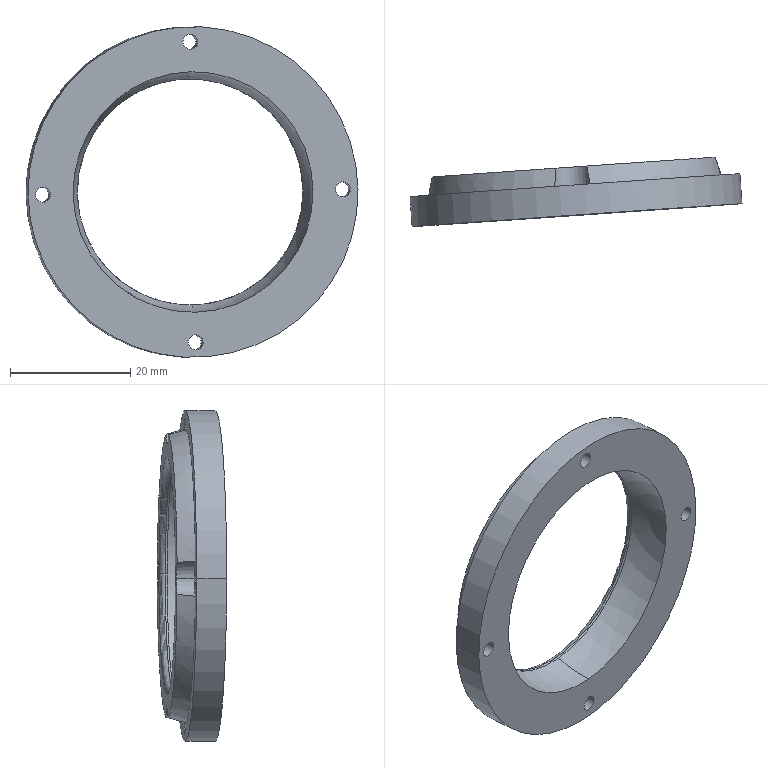Component | SolidWorks | ClampingMechanism-1_BallJointFixed-1 | 1 solid | 28 faces | box 55.21 x 11.53 x 55 mm | volume 7588 mm3 | cylinder 15 | sphere 6 | torus 4 | plane 3 | commonest cylinder face diameters 2.5 x8 6 x5 55 x2
STEP:
#1=COLOUR_RGB('',0.7922,0.8196,0.9333);
#2=FILL_AREA_STYLE_COLOUR('',#1);
#3=FILL_AREA_STYLE('',(#2));
#4=SURFACE_STYLE_FILL_AREA(#3);
#5=SURFACE_SIDE_STYLE('',(#4));
#6=SURFACE_STYLE_USAGE(.BOTH.,#5);
#7=PRESENTATION_STYLE_ASSIGNMENT((#6));
#8=CARTESIAN_POINT('',(1.976,-7.995,-21.39));
#9=VERTEX_POINT('',#8);
#10=CARTESIAN_POINT('',(1.934,-7.959,-21.391));
#11=VERTEX_POINT('',#10);
#12=CARTESIAN_POINT('',(1.937,-7.998,-21.391));
#13=DIRECTION('',(-0.01767,-0.001232,0.9998));
#14=DIRECTION('',(0.9998,0.,0.01767));
#15=AXIS2_PLACEMENT_3D('',#12,#13,#14);
#16=CIRCLE('',#15,0.03937);
#17=EDGE_CURVE('',#9,#11,#16,.T.);
#18=ORIENTED_EDGE('',*,*,#17,.F.);
#19=CARTESIAN_POINT('',(3.452,-7.892,-21.364));
#20=VERTEX_POINT('',#19);
#21=CARTESIAN_POINT('',(2.714,-7.944,-21.377));
#22=DIRECTION('',(0.06956,-0.9976,-0.));
#23=DIRECTION('',(0.9976,0.06956,0.));
#24=AXIS2_PLACEMENT_3D('',#21,#22,#23);
#25=CIRCLE('',#24,0.7401);
#26=EDGE_CURVE('',#9,#20,#25,.T.);
#27=ORIENTED_EDGE('',*,*,#26,.T.);
#28=CARTESIAN_POINT('',(3.489,-7.85,-21.363));
#29=VERTEX_POINT('',#28);
#30=CARTESIAN_POINT('',(3.492,-7.89,-21.363));
#31=DIRECTION('',(0.01767,0.001232,-0.9998));
#32=DIRECTION('',(-0.9998,0.,-0.01767));
#33=AXIS2_PLACEMENT_3D('',#30,#31,#32);
#34=CIRCLE('',#33,0.03937);
#35=EDGE_CURVE('',#20,#29,#34,.T.);
#36=ORIENTED_EDGE('',*,*,#35,.T.);
#37=CARTESIAN_POINT('',(2.711,-7.905,-21.377));
#38=DIRECTION('',(0.06956,-0.9976,-0.));
#39=DIRECTION('',(0.9974,0.06955,0.01772));
#40=AXIS2_PLACEMENT_3D('',#37,#38,#39);
#41=CIRCLE('',#40,0.7795);
#42=EDGE_CURVE('',#11,#29,#41,.T.);
#43=ORIENTED_EDGE('',*,*,#42,.F.);
#44=EDGE_LOOP('',(#18,#27,#36,#43));
#45=FACE_OUTER_BOUND('',#44,.T.);
#46=CARTESIAN_POINT('',(2.714,-7.944,-21.377));
#47=DIRECTION('',(0.06956,-0.9976,-0.));
#48=DIRECTION('',(0.9974,0.06955,0.01772));
#49=AXIS2_PLACEMENT_3D('',#46,#47,#48);
#50=TOROIDAL_SURFACE('',#49,0.7795,0.03937);
#51=ADVANCED_FACE('',(#45),#50,.T.);
#52=ORIENTED_EDGE('',*,*,#35,.F.);
#53=CARTESIAN_POINT('',(2.714,-7.944,-21.377));
#54=DIRECTION('',(0.06956,-0.9976,-0.));
#55=DIRECTION('',(0.9976,0.06956,0.));
#56=AXIS2_PLACEMENT_3D('',#53,#54,#55);
#57=CIRCLE('',#56,0.7401);
#58=EDGE_CURVE('',#20,#9,#57,.T.);
#59=ORIENTED_EDGE('',*,*,#58,.T.);
#60=ORIENTED_EDGE('',*,*,#17,.T.);
#61=CARTESIAN_POINT('',(2.711,-7.905,-21.377));
#62=DIRECTION('',(0.06956,-0.9976,-0.));
#63=DIRECTION('',(0.9974,0.06955,0.01772));
#64=AXIS2_PLACEMENT_3D('',#61,#62,#63);
#65=CIRCLE('',#64,0.7795);
#66=EDGE_CURVE('',#29,#11,#65,.T.);
#67=ORIENTED_EDGE('',*,*,#66,.F.);
#68=EDGE_LOOP('',(#52,#59,#60,#67));
#69=FACE_OUTER_BOUND('',#68,.T.);
#70=CARTESIAN_POINT('',(2.714,-7.944,-21.377));
#71=DIRECTION('',(0.06956,-0.9976,-0.));
#72=DIRECTION('',(0.9974,0.06955,0.01772));
#73=AXIS2_PLACEMENT_3D('',#70,#71,#72);
#74=TOROIDAL_SURFACE('',#73,0.7795,0.03937);
#75=ADVANCED_FACE('',(#69),#74,.T.);
#76=ORIENTED_EDGE('',*,*,#58,.F.);
#77=CARTESIAN_POINT('',(3.456,-7.905,-21.364));
#78=VERTEX_POINT('',#77);
#79=CARTESIAN_POINT('',(3.492,-7.89,-21.363));
#80=DIRECTION('',(0.01767,0.001232,-0.9998));
#81=DIRECTION('',(-0.9998,0.,-0.01767));
#82=AXIS2_PLACEMENT_3D('',#79,#80,#81);
#83=CIRCLE('',#82,0.03937);
#84=EDGE_CURVE('',#78,#20,#83,.T.);
#85=ORIENTED_EDGE('',*,*,#84,.F.);
#86=CARTESIAN_POINT('',(2.702,-7.958,-20.635));
#87=VERTEX_POINT('',#86);
#88=CARTESIAN_POINT('',(2.715,-7.957,-21.377));
#89=DIRECTION('',(-0.06956,0.9976,0.));
#90=DIRECTION('',(0.9974,0.06955,0.01772));
#91=AXIS2_PLACEMENT_3D('',#88,#89,#90);
#92=CIRCLE('',#91,0.7424);
#93=EDGE_CURVE('',#87,#78,#92,.T.);
#94=ORIENTED_EDGE('',*,*,#93,.F.);
#95=CARTESIAN_POINT('',(1.975,-8.009,-21.39));
#96=VERTEX_POINT('',#95);
#97=CARTESIAN_POINT('',(2.715,-7.957,-21.377));
#98=DIRECTION('',(-0.06956,0.9976,0.));
#99=DIRECTION('',(0.9974,0.06955,0.01772));
#100=AXIS2_PLACEMENT_3D('',#97,#98,#99);
#101=CIRCLE('',#100,0.7424);
#102=EDGE_CURVE('',#96,#87,#101,.T.);
#103=ORIENTED_EDGE('',*,*,#102,.F.);
#104=CARTESIAN_POINT('',(1.937,-7.998,-21.391));
#105=DIRECTION('',(-0.01767,-0.001232,0.9998));
#106=DIRECTION('',(0.9998,0.,0.01767));
#107=AXIS2_PLACEMENT_3D('',#104,#105,#106);
#108=CIRCLE('',#107,0.03937);
#109=EDGE_CURVE('',#96,#9,#108,.T.);
#110=ORIENTED_EDGE('',*,*,#109,.T.);
#111=EDGE_LOOP('',(#76,#85,#94,#103,#110));
#112=FACE_OUTER_BOUND('',#111,.T.);
#113=CARTESIAN_POINT('',(2.714,-7.944,-21.377));
#114=DIRECTION('',(0.06956,-0.9976,-0.));
#115=DIRECTION('',(0.9974,0.06955,0.01772));
#116=AXIS2_PLACEMENT_3D('',#113,#114,#115);
#117=TOROIDAL_SURFACE('',#116,0.7795,0.03937);
#118=ADVANCED_FACE('',(#112),#117,.T.);
#119=CARTESIAN_POINT('',(1.848,-7.965,-21.392));
#120=VERTEX_POINT('',#119);
#121=CARTESIAN_POINT('',(1.785,-7.969,-21.29));
#122=VERTEX_POINT('',#121);
#123=CARTESIAN_POINT('',(1.73,-7.973,-21.394));
#124=DIRECTION('',(0.06956,-0.9976,-0.));
#125=DIRECTION('',(0.9974,0.06955,0.01772));
#126=AXIS2_PLACEMENT_3D('',#123,#124,#125);
#127=CIRCLE('',#126,0.1181);
#128=EDGE_CURVE('',#120,#122,#127,.T.);
#129=ORIENTED_EDGE('',*,*,#128,.F.);
#130=CARTESIAN_POINT('',(1.856,-8.083,-21.392));
#131=VERTEX_POINT('',#130);
#132=CARTESIAN_POINT('',(1.828,-7.69,-21.392));
#133=DIRECTION('',(0.06956,-0.9976,-0.));
#134=VECTOR('',#133,39.37);
#135=LINE('',#132,#134);
#136=EDGE_CURVE('',#120,#131,#135,.T.);
#137=ORIENTED_EDGE('',*,*,#136,.T.);
#138=CARTESIAN_POINT('',(1.763,-8.089,-21.279));
#139=VERTEX_POINT('',#138);
#140=CARTESIAN_POINT('',(1.738,-8.091,-21.394));
#141=DIRECTION('',(-0.06956,0.9976,0.));
#142=DIRECTION('',(-0.9974,-0.06955,-0.01772));
#143=AXIS2_PLACEMENT_3D('',#140,#141,#142);
#144=CIRCLE('',#143,0.1181);
#145=EDGE_CURVE('',#139,#131,#144,.T.);
#146=ORIENTED_EDGE('',*,*,#145,.F.);
#147=CARTESIAN_POINT('',(1.763,-8.089,-21.279));
#148=CARTESIAN_POINT('',(1.768,-8.048,-21.28));
#149=CARTESIAN_POINT('',(1.776,-8.008,-21.283));
#150=CARTESIAN_POINT('',(1.785,-7.969,-21.29));
#151=B_SPLINE_CURVE_WITH_KNOTS('',3,(#147,#148,#149,#150),.UNSPECIFIED.,.F.,.F.,(4,4),(0.0000002,0.003113),.UNSPECIFIED.);
#152=EDGE_CURVE('',#139,#122,#151,.T.);
#153=ORIENTED_EDGE('',*,*,#152,.T.);
#154=EDGE_LOOP('',(#129,#137,#146,#153));
#155=FACE_OUTER_BOUND('',#154,.T.);
#156=CARTESIAN_POINT('',(1.711,-7.698,-21.394));
#157=DIRECTION('',(0.06956,-0.9976,-0.));
#158=DIRECTION('',(0.9974,0.06955,0.01772));
#159=AXIS2_PLACEMENT_3D('',#156,#157,#158);
#160=CYLINDRICAL_SURFACE('',#159,0.1181);
#161=ADVANCED_FACE('',(#155),#160,.F.);
#162=ORIENTED_EDGE('',*,*,#93,.T.);
#163=CARTESIAN_POINT('',(2.728,-7.956,-22.119));
#164=VERTEX_POINT('',#163);
#165=CARTESIAN_POINT('',(2.715,-7.957,-21.377));
#166=DIRECTION('',(-0.06956,0.9976,0.));
#167=DIRECTION('',(0.9974,0.06955,0.01772));
#168=AXIS2_PLACEMENT_3D('',#165,#166,#167);
#169=CIRCLE('',#168,0.7424);
#170=EDGE_CURVE('',#78,#164,#169,.T.);
#171=ORIENTED_EDGE('',*,*,#170,.T.);
#172=CARTESIAN_POINT('',(2.747,-8.218,-22.164));
#173=VERTEX_POINT('',#172);
#174=CARTESIAN_POINT('',(2.733,-8.219,-21.377));
#175=DIRECTION('',(-0.9974,-0.06955,-0.01772));
#176=DIRECTION('',(0.06956,-0.9976,0.));
#177=AXIS2_PLACEMENT_3D('',#174,#175,#176);
#178=CIRCLE('',#177,0.7874);
#179=EDGE_CURVE('',#164,#173,#178,.T.);
#180=ORIENTED_EDGE('',*,*,#179,.T.);
#181=CARTESIAN_POINT('',(2.719,-8.22,-20.589));
#182=VERTEX_POINT('',#181);
#183=CARTESIAN_POINT('',(2.733,-8.219,-21.377));
#184=DIRECTION('',(-0.06956,0.9976,0.));
#185=DIRECTION('',(0.9974,0.06955,0.01772));
#186=AXIS2_PLACEMENT_3D('',#183,#184,#185);
#187=CIRCLE('',#186,0.7874);
#188=EDGE_CURVE('',#182,#173,#187,.T.);
#189=ORIENTED_EDGE('',*,*,#188,.F.);
#190=CARTESIAN_POINT('',(2.733,-8.219,-21.377));
#191=DIRECTION('',(0.9974,0.06955,0.01772));
#192=DIRECTION('',(-0.06956,0.9976,0.));
#193=AXIS2_PLACEMENT_3D('',#190,#191,#192);
#194=CIRCLE('',#193,0.7874);
#195=EDGE_CURVE('',#87,#182,#194,.T.);
#196=ORIENTED_EDGE('',*,*,#195,.F.);
#197=EDGE_LOOP('',(#162,#171,#180,#189,#196));
#198=FACE_OUTER_BOUND('',#197,.T.);
#199=CARTESIAN_POINT('',(2.733,-8.219,-21.377));
#200=DIRECTION('',(-0.9974,-0.06955,-0.01772));
#201=DIRECTION('',(-0.01767,-0.001232,0.9998));
#202=AXIS2_PLACEMENT_3D('',#199,#200,#201);
#203=SPHERICAL_SURFACE('',#202,0.7874);
#204=ADVANCED_FACE('',(#198),#203,.F.);
#205=CARTESIAN_POINT('',(3.8,-7.947,-21.358));
#206=VERTEX_POINT('',#205);
#207=CARTESIAN_POINT('',(1.64,-8.098,-21.396));
#208=VERTEX_POINT('',#207);
#209=CARTESIAN_POINT('',(2.72,-8.022,-21.377));
#210=DIRECTION('',(0.06956,-0.9976,-0.));
#211=DIRECTION('',(0.9974,0.06955,0.01772));
#212=AXIS2_PLACEMENT_3D('',#209,#210,#211);
#213=CIRCLE('',#212,1.083);
#214=EDGE_CURVE('',#206,#208,#213,.T.);
#215=ORIENTED_EDGE('',*,*,#214,.T.);
#216=CARTESIAN_POINT('',(1.653,-8.294,-21.396));
#217=VERTEX_POINT('',#216);
#218=CARTESIAN_POINT('',(1.64,-8.098,-21.396));
#219=DIRECTION('',(0.06956,-0.9976,-0.));
#220=VECTOR('',#219,39.37);
#221=LINE('',#218,#220);
#222=EDGE_CURVE('',#208,#217,#221,.T.);
#223=ORIENTED_EDGE('',*,*,#222,.T.);
#224=CARTESIAN_POINT('',(3.813,-8.144,-21.358));
#225=VERTEX_POINT('',#224);
#226=CARTESIAN_POINT('',(2.733,-8.219,-21.377));
#227=DIRECTION('',(0.06956,-0.9976,-0.));
#228=DIRECTION('',(0.9974,0.06955,0.01772));
#229=AXIS2_PLACEMENT_3D('',#226,#227,#228);
#230=CIRCLE('',#229,1.083);
#231=EDGE_CURVE('',#225,#217,#230,.T.);
#232=ORIENTED_EDGE('',*,*,#231,.F.);
#233=CARTESIAN_POINT('',(3.8,-7.947,-21.358));
#234=DIRECTION('',(0.06956,-0.9976,-0.));
#235=VECTOR('',#234,39.37);
#236=LINE('',#233,#235);
#237=EDGE_CURVE('',#206,#225,#236,.T.);
#238=ORIENTED_EDGE('',*,*,#237,.F.);
#239=EDGE_LOOP('',(#215,#223,#232,#238));
#240=FACE_OUTER_BOUND('',#239,.T.);
#241=CARTESIAN_POINT('',(2.72,-8.022,-21.377));
#242=DIRECTION('',(0.06956,-0.9976,-0.));
#243=DIRECTION('',(0.9974,0.06955,0.01772));
#244=AXIS2_PLACEMENT_3D('',#241,#242,#243);
#245=CYLINDRICAL_SURFACE('',#244,1.083);
#246=ADVANCED_FACE('',(#240),#245,.T.);
#247=CARTESIAN_POINT('',(1.689,-8.094,-21.395));
#248=VERTEX_POINT('',#247);
#249=CARTESIAN_POINT('',(1.787,-8.087,-21.393));
#250=VERTEX_POINT('',#249);
#251=CARTESIAN_POINT('',(1.738,-8.091,-21.394));
#252=DIRECTION('',(0.06956,-0.9976,-0.));
#253=DIRECTION('',(0.9974,0.06955,0.01772));
#254=AXIS2_PLACEMENT_3D('',#251,#252,#253);
#255=CIRCLE('',#254,0.04921);
#256=EDGE_CURVE('',#248,#250,#255,.T.);
#257=ORIENTED_EDGE('',*,*,#256,.F.);
#258=CARTESIAN_POINT('',(1.703,-8.291,-21.395));
#259=VERTEX_POINT('',#258);
#260=CARTESIAN_POINT('',(1.703,-8.291,-21.395));
#261=DIRECTION('',(0.06956,-0.9976,-0.));
#262=VECTOR('',#261,39.37);
#263=LINE('',#260,#262);
#264=EDGE_CURVE('',#248,#259,#263,.T.);
#265=ORIENTED_EDGE('',*,*,#264,.T.);
#266=CARTESIAN_POINT('',(1.801,-8.284,-21.393));
#267=VERTEX_POINT('',#266);
#268=CARTESIAN_POINT('',(1.752,-8.287,-21.394));
#269=DIRECTION('',(0.06956,-0.9976,-0.));
#270=DIRECTION('',(0.9974,0.06955,0.01772));
#271=AXIS2_PLACEMENT_3D('',#268,#269,#270);
#272=CIRCLE('',#271,0.04921);
#273=EDGE_CURVE('',#259,#267,#272,.T.);
#274=ORIENTED_EDGE('',*,*,#273,.T.);
#275=CARTESIAN_POINT('',(1.801,-8.284,-21.393));
#276=DIRECTION('',(0.06956,-0.9976,-0.));
#277=VECTOR('',#276,39.37);
#278=LINE('',#275,#277);
#279=EDGE_CURVE('',#250,#267,#278,.T.);
#280=ORIENTED_EDGE('',*,*,#279,.F.);
#281=EDGE_LOOP('',(#257,#265,#274,#280));
#282=FACE_OUTER_BOUND('',#281,.T.);
#283=CARTESIAN_POINT('',(1.752,-8.287,-21.394));
#284=DIRECTION('',(0.06956,-0.9976,-0.));
#285=DIRECTION('',(0.9974,0.06955,0.01772));
#286=AXIS2_PLACEMENT_3D('',#283,#284,#285);
#287=CYLINDRICAL_SURFACE('',#286,0.04921);
#288=ADVANCED_FACE('',(#282),#287,.F.);
#289=CARTESIAN_POINT('',(2.653,-8.027,-20.394));
#290=VERTEX_POINT('',#289);
#291=CARTESIAN_POINT('',(2.751,-8.02,-20.392));
#292=VERTEX_POINT('',#291);
#293=CARTESIAN_POINT('',(2.702,-8.024,-20.393));
#294=DIRECTION('',(0.06956,-0.9976,-0.));
#295=DIRECTION('',(0.9974,0.06955,0.01772));
#296=AXIS2_PLACEMENT_3D('',#293,#294,#295);
#297=CIRCLE('',#296,0.04921);
#298=EDGE_CURVE('',#290,#292,#297,.T.);
#299=ORIENTED_EDGE('',*,*,#298,.F.);
#300=CARTESIAN_POINT('',(2.667,-8.223,-20.394));
#301=VERTEX_POINT('',#300);
#302=CARTESIAN_POINT('',(2.667,-8.223,-20.394));
#303=DIRECTION('',(0.06956,-0.9976,-0.));
#304=VECTOR('',#303,39.37);
#305=LINE('',#302,#304);
#306=EDGE_CURVE('',#290,#301,#305,.T.);
#307=ORIENTED_EDGE('',*,*,#306,.T.);
#308=CARTESIAN_POINT('',(2.765,-8.217,-20.392));
#309=VERTEX_POINT('',#308);
#310=CARTESIAN_POINT('',(2.716,-8.22,-20.393));
#311=DIRECTION('',(0.06956,-0.9976,-0.));
#312=DIRECTION('',(0.9974,0.06955,0.01772));
#313=AXIS2_PLACEMENT_3D('',#310,#311,#312);
#314=CIRCLE('',#313,0.04921);
#315=EDGE_CURVE('',#301,#309,#314,.T.);
#316=ORIENTED_EDGE('',*,*,#315,.T.);
#317=CARTESIAN_POINT('',(2.765,-8.217,-20.392));
#318=DIRECTION('',(0.06956,-0.9976,-0.));
#319=VECTOR('',#318,39.37);
#320=LINE('',#317,#319);
#321=EDGE_CURVE('',#292,#309,#320,.T.);
#322=ORIENTED_EDGE('',*,*,#321,.F.);
#323=EDGE_LOOP('',(#299,#307,#316,#322));
#324=FACE_OUTER_BOUND('',#323,.T.);
#325=CARTESIAN_POINT('',(2.716,-8.22,-20.393));
#326=DIRECTION('',(0.06956,-0.9976,-0.));
#327=DIRECTION('',(0.9974,0.06955,0.01772));
#328=AXIS2_PLACEMENT_3D('',#325,#326,#327);
#329=CYLINDRICAL_SURFACE('',#328,0.04921);
#330=ADVANCED_FACE('',(#324),#329,.F.);
#331=CARTESIAN_POINT('',(3.652,-7.957,-21.36));
#332=VERTEX_POINT('',#331);
#333=CARTESIAN_POINT('',(3.75,-7.951,-21.358));
#334=VERTEX_POINT('',#333);
#335=CARTESIAN_POINT('',(3.701,-7.954,-21.359));
#336=DIRECTION('',(0.06956,-0.9976,-0.));
#337=DIRECTION('',(0.9974,0.06955,0.01772));
#338=AXIS2_PLACEMENT_3D('',#335,#336,#337);
#339=CIRCLE('',#338,0.04921);
#340=EDGE_CURVE('',#332,#334,#339,.T.);
#341=ORIENTED_EDGE('',*,*,#340,.F.);
#342=CARTESIAN_POINT('',(3.666,-8.154,-21.36));
#343=VERTEX_POINT('',#342);
#344=CARTESIAN_POINT('',(3.666,-8.154,-21.36));
#345=DIRECTION('',(0.06956,-0.9976,-0.));
#346=VECTOR('',#345,39.37);
#347=LINE('',#344,#346);
#348=EDGE_CURVE('',#332,#343,#347,.T.);
#349=ORIENTED_EDGE('',*,*,#348,.T.);
#350=CARTESIAN_POINT('',(3.764,-8.147,-21.358));
#351=VERTEX_POINT('',#350);
#352=CARTESIAN_POINT('',(3.715,-8.15,-21.359));
#353=DIRECTION('',(0.06956,-0.9976,-0.));
#354=DIRECTION('',(0.9974,0.06955,0.01772));
#355=AXIS2_PLACEMENT_3D('',#352,#353,#354);
#356=CIRCLE('',#355,0.04921);
#357=EDGE_CURVE('',#343,#351,#356,.T.);
#358=ORIENTED_EDGE('',*,*,#357,.T.);
#359=CARTESIAN_POINT('',(3.764,-8.147,-21.358));
#360=DIRECTION('',(0.06956,-0.9976,-0.));
#361=VECTOR('',#360,39.37);
#362=LINE('',#359,#361);
#363=EDGE_CURVE('',#334,#351,#362,.T.);
#364=ORIENTED_EDGE('',*,*,#363,.F.);
#365=EDGE_LOOP('',(#341,#349,#358,#364));
#366=FACE_OUTER_BOUND('',#365,.T.);
#367=CARTESIAN_POINT('',(3.715,-8.15,-21.359));
#368=DIRECTION('',(0.06956,-0.9976,-0.));
#369=DIRECTION('',(0.9974,0.06955,0.01772));
#370=AXIS2_PLACEMENT_3D('',#367,#368,#369);
#371=CYLINDRICAL_SURFACE('',#370,0.04921);
#372=ADVANCED_FACE('',(#366),#371,.F.);
#373=CARTESIAN_POINT('',(2.688,-8.025,-22.362));
#374=VERTEX_POINT('',#373);
#375=CARTESIAN_POINT('',(2.786,-8.018,-22.36));
#376=VERTEX_POINT('',#375);
#377=CARTESIAN_POINT('',(2.737,-8.021,-22.361));
#378=DIRECTION('',(0.06956,-0.9976,-0.));
#379=DIRECTION('',(0.9974,0.06955,0.01772));
#380=AXIS2_PLACEMENT_3D('',#377,#378,#379);
#381=CIRCLE('',#380,0.04921);
#382=EDGE_CURVE('',#374,#376,#381,.T.);
#383=ORIENTED_EDGE('',*,*,#382,.F.);
#384=CARTESIAN_POINT('',(2.702,-8.221,-22.362));
#385=VERTEX_POINT('',#384);
#386=CARTESIAN_POINT('',(2.702,-8.221,-22.362));
#387=DIRECTION('',(0.06956,-0.9976,-0.));
#388=VECTOR('',#387,39.37);
#389=LINE('',#386,#388);
#390=EDGE_CURVE('',#374,#385,#389,.T.);
#391=ORIENTED_EDGE('',*,*,#390,.T.);
#392=CARTESIAN_POINT('',(2.8,-8.214,-22.36));
#393=VERTEX_POINT('',#392);
#394=CARTESIAN_POINT('',(2.751,-8.218,-22.361));
#395=DIRECTION('',(0.06956,-0.9976,-0.));
#396=DIRECTION('',(0.9974,0.06955,0.01772));
#397=AXIS2_PLACEMENT_3D('',#394,#395,#396);
#398=CIRCLE('',#397,0.04921);
#399=EDGE_CURVE('',#385,#393,#398,.T.);
#400=ORIENTED_EDGE('',*,*,#399,.T.);
#401=CARTESIAN_POINT('',(2.8,-8.214,-22.36));
#402=DIRECTION('',(0.06956,-0.9976,-0.));
#403=VECTOR('',#402,39.37);
#404=LINE('',#401,#403);
#405=EDGE_CURVE('',#376,#393,#404,.T.);
#406=ORIENTED_EDGE('',*,*,#405,.F.);
#407=EDGE_LOOP('',(#383,#391,#400,#406));
#408=FACE_OUTER_BOUND('',#407,.T.);
#409=CARTESIAN_POINT('',(2.751,-8.218,-22.361));
#410=DIRECTION('',(0.06956,-0.9976,-0.));
#411=DIRECTION('',(0.9974,0.06955,0.01772));
#412=AXIS2_PLACEMENT_3D('',#409,#410,#411);
#413=CYLINDRICAL_SURFACE('',#412,0.04921);
#414=ADVANCED_FACE('',(#408),#413,.F.);
#415=CARTESIAN_POINT('',(3.634,-7.84,-21.257));
#416=VERTEX_POINT('',#415);
#417=CARTESIAN_POINT('',(3.673,-7.956,-21.245));
#418=VERTEX_POINT('',#417);
#419=CARTESIAN_POINT('',(3.634,-7.84,-21.257));
#420=CARTESIAN_POINT('',(3.649,-7.878,-21.25));
#421=CARTESIAN_POINT('',(3.662,-7.916,-21.247));
#422=CARTESIAN_POINT('',(3.673,-7.956,-21.245));
#423=B_SPLINE_CURVE_WITH_KNOTS('',3,(#419,#420,#421,#422),.UNSPECIFIED.,.F.,.F.,(4,4),(0.01359,0.01671),.UNSPECIFIED.);
#424=EDGE_CURVE('',#416,#418,#423,.T.);
#425=ORIENTED_EDGE('',*,*,#424,.F.);
#426=CARTESIAN_POINT('',(2.798,-7.899,-20.448));
#427=VERTEX_POINT('',#426);
#428=CARTESIAN_POINT('',(2.711,-7.905,-21.377));
#429=DIRECTION('',(0.06956,-0.9976,-0.));
#430=DIRECTION('',(0.9974,0.06955,0.01772));
#431=AXIS2_PLACEMENT_3D('',#428,#429,#430);
#432=CIRCLE('',#431,0.9325);
#433=EDGE_CURVE('',#416,#427,#432,.T.);
#434=ORIENTED_EDGE('',*,*,#433,.T.);
#435=CARTESIAN_POINT('',(2.817,-8.016,-20.417));
#436=VERTEX_POINT('',#435);
#437=CARTESIAN_POINT('',(2.817,-8.016,-20.417));
#438=CARTESIAN_POINT('',(2.813,-7.976,-20.425));
#439=CARTESIAN_POINT('',(2.807,-7.936,-20.436));
#440=CARTESIAN_POINT('',(2.798,-7.899,-20.448));
#441=B_SPLINE_CURVE_WITH_KNOTS('',3,(#437,#438,#439,#440),.UNSPECIFIED.,.F.,.F.,(4,4),(0.0000002,0.003113),.UNSPECIFIED.);
#442=EDGE_CURVE('',#436,#427,#441,.T.);
#443=ORIENTED_EDGE('',*,*,#442,.F.);
#444=CARTESIAN_POINT('',(2.72,-8.022,-21.377));
#445=DIRECTION('',(0.06956,-0.9976,-0.));
#446=DIRECTION('',(0.9974,0.06955,0.01772));
#447=AXIS2_PLACEMENT_3D('',#444,#445,#446);
#448=CIRCLE('',#447,0.9644);
#449=EDGE_CURVE('',#418,#436,#448,.T.);
#450=ORIENTED_EDGE('',*,*,#449,.F.);
#451=EDGE_LOOP('',(#425,#434,#443,#450));
#452=FACE_OUTER_BOUND('',#451,.T.);
#453=CARTESIAN_POINT('',(2.733,-8.219,-21.377));
#454=DIRECTION('',(-0.9974,-0.06955,-0.01772));
#455=DIRECTION('',(-0.01767,-0.001232,0.9998));
#456=AXIS2_PLACEMENT_3D('',#453,#454,#455);
#457=SPHERICAL_SURFACE('',#456,0.9843);
#458=ADVANCED_FACE('',(#452),#457,.T.);
#459=CARTESIAN_POINT('',(2.592,-7.913,-20.452));
#460=VERTEX_POINT('',#459);
#461=CARTESIAN_POINT('',(2.588,-8.032,-20.421));
#462=VERTEX_POINT('',#461);
#463=CARTESIAN_POINT('',(2.592,-7.913,-20.452));
#464=CARTESIAN_POINT('',(2.588,-7.952,-20.44));
#465=CARTESIAN_POINT('',(2.587,-7.991,-20.429));
#466=CARTESIAN_POINT('',(2.588,-8.032,-20.421));
#467=B_SPLINE_CURVE_WITH_KNOTS('',3,(#463,#464,#465,#466),.UNSPECIFIED.,.F.,.F.,(4,4),(0.01359,0.01671),.UNSPECIFIED.);
#468=EDGE_CURVE('',#460,#462,#467,.T.);
#469=ORIENTED_EDGE('',*,*,#468,.F.);
#470=CARTESIAN_POINT('',(2.711,-7.905,-21.377));
#471=DIRECTION('',(0.06956,-0.9976,-0.));
#472=DIRECTION('',(0.9974,0.06955,0.01772));
#473=AXIS2_PLACEMENT_3D('',#470,#471,#472);
#474=CIRCLE('',#473,0.9325);
#475=EDGE_CURVE('',#460,#122,#474,.T.);
#476=ORIENTED_EDGE('',*,*,#475,.T.);
#477=ORIENTED_EDGE('',*,*,#152,.F.);
#478=CARTESIAN_POINT('',(2.72,-8.022,-21.377));
#479=DIRECTION('',(0.06956,-0.9976,-0.));
#480=DIRECTION('',(0.9974,0.06955,0.01772));
#481=AXIS2_PLACEMENT_3D('',#478,#479,#480);
#482=CIRCLE('',#481,0.9644);
#483=EDGE_CURVE('',#462,#139,#482,.T.);
#484=ORIENTED_EDGE('',*,*,#483,.F.);
#485=EDGE_LOOP('',(#469,#476,#477,#484));
#486=FACE_OUTER_BOUND('',#485,.T.);
#487=CARTESIAN_POINT('',(2.733,-8.219,-21.377));
#488=DIRECTION('',(-0.9974,-0.06955,-0.01772));
#489=DIRECTION('',(-0.01767,-0.001232,0.9998));
#490=AXIS2_PLACEMENT_3D('',#487,#488,#489);
#491=SPHERICAL_SURFACE('',#490,0.9843);
#492=ADVANCED_FACE('',(#486),#491,.T.);
#493=CARTESIAN_POINT('',(1.789,-7.969,-21.496));
#494=VERTEX_POINT('',#493);
#495=CARTESIAN_POINT('',(1.767,-8.089,-21.509));
#496=VERTEX_POINT('',#495);
#497=CARTESIAN_POINT('',(1.789,-7.969,-21.496));
#498=CARTESIAN_POINT('',(1.779,-8.008,-21.503));
#499=CARTESIAN_POINT('',(1.772,-8.048,-21.507));
#500=CARTESIAN_POINT('',(1.767,-8.089,-21.509));
#501=B_SPLINE_CURVE_WITH_KNOTS('',3,(#497,#498,#499,#500),.UNSPECIFIED.,.F.,.F.,(4,4),(0.01359,0.01671),.UNSPECIFIED.);
#502=EDGE_CURVE('',#494,#496,#501,.T.);
#503=ORIENTED_EDGE('',*,*,#502,.F.);
#504=CARTESIAN_POINT('',(2.625,-7.911,-22.305));
#505=VERTEX_POINT('',#504);
#506=CARTESIAN_POINT('',(2.711,-7.905,-21.377));
#507=DIRECTION('',(0.06956,-0.9976,-0.));
#508=DIRECTION('',(0.9974,0.06955,0.01772));
#509=AXIS2_PLACEMENT_3D('',#506,#507,#508);
#510=CIRCLE('',#509,0.9325);
#511=EDGE_CURVE('',#494,#505,#510,.T.);
#512=ORIENTED_EDGE('',*,*,#511,.T.);
#513=CARTESIAN_POINT('',(2.622,-8.029,-22.336));
#514=VERTEX_POINT('',#513);
#515=CARTESIAN_POINT('',(2.622,-8.029,-22.336));
#516=CARTESIAN_POINT('',(2.621,-7.989,-22.328));
#517=CARTESIAN_POINT('',(2.621,-7.949,-22.318));
#518=CARTESIAN_POINT('',(2.625,-7.911,-22.305));
#519=B_SPLINE_CURVE_WITH_KNOTS('',3,(#515,#516,#517,#518),.UNSPECIFIED.,.F.,.F.,(4,4),(0.0000002,0.003113),.UNSPECIFIED.);
#520=EDGE_CURVE('',#514,#505,#519,.T.);
#521=ORIENTED_EDGE('',*,*,#520,.F.);
#522=CARTESIAN_POINT('',(2.72,-8.022,-21.377));
#523=DIRECTION('',(0.06956,-0.9976,-0.));
#524=DIRECTION('',(0.9974,0.06955,0.01772));
#525=AXIS2_PLACEMENT_3D('',#522,#523,#524);
#526=CIRCLE('',#525,0.9644);
#527=EDGE_CURVE('',#496,#514,#526,.T.);
#528=ORIENTED_EDGE('',*,*,#527,.F.);
#529=EDGE_LOOP('',(#503,#512,#521,#528));
#530=FACE_OUTER_BOUND('',#529,.T.);
#531=CARTESIAN_POINT('',(2.733,-8.219,-21.377));
#532=DIRECTION('',(-0.9974,-0.06955,-0.01772));
#533=DIRECTION('',(-0.01767,-0.001232,0.9998));
#534=AXIS2_PLACEMENT_3D('',#531,#532,#533);
#535=SPHERICAL_SURFACE('',#534,0.9843);
#536=ADVANCED_FACE('',(#530),#535,.T.);
#537=CARTESIAN_POINT('',(2.831,-7.896,-22.302));
#538=VERTEX_POINT('',#537);
#539=CARTESIAN_POINT('',(2.851,-8.013,-22.332));
#540=VERTEX_POINT('',#539);
#541=CARTESIAN_POINT('',(2.831,-7.896,-22.302));
#542=CARTESIAN_POINT('',(2.84,-7.934,-22.314));
#543=CARTESIAN_POINT('',(2.846,-7.973,-22.324));
#544=CARTESIAN_POINT('',(2.851,-8.013,-22.332));
#545=B_SPLINE_CURVE_WITH_KNOTS('',3,(#541,#542,#543,#544),.UNSPECIFIED.,.F.,.F.,(4,4),(0.01359,0.01671),.UNSPECIFIED.);
#546=EDGE_CURVE('',#538,#540,#545,.T.);
#547=ORIENTED_EDGE('',*,*,#546,.F.);
#548=CARTESIAN_POINT('',(3.638,-7.84,-21.464));
#549=VERTEX_POINT('',#548);
#550=CARTESIAN_POINT('',(2.711,-7.905,-21.377));
#551=DIRECTION('',(0.06956,-0.9976,-0.));
#552=DIRECTION('',(0.9974,0.06955,0.01772));
#553=AXIS2_PLACEMENT_3D('',#550,#551,#552);
#554=CIRCLE('',#553,0.9325);
#555=EDGE_CURVE('',#538,#549,#554,.T.);
#556=ORIENTED_EDGE('',*,*,#555,.T.);
#557=CARTESIAN_POINT('',(3.677,-7.956,-21.475));
#558=VERTEX_POINT('',#557);
#559=CARTESIAN_POINT('',(3.677,-7.956,-21.475));
#560=CARTESIAN_POINT('',(3.666,-7.916,-21.473));
#561=CARTESIAN_POINT('',(3.653,-7.878,-21.47));
#562=CARTESIAN_POINT('',(3.638,-7.84,-21.464));
#563=B_SPLINE_CURVE_WITH_KNOTS('',3,(#559,#560,#561,#562),.UNSPECIFIED.,.F.,.F.,(4,4),(0.0000002,0.003113),.UNSPECIFIED.);
#564=EDGE_CURVE('',#558,#549,#563,.T.);
#565=ORIENTED_EDGE('',*,*,#564,.F.);
#566=CARTESIAN_POINT('',(2.72,-8.022,-21.377));
#567=DIRECTION('',(0.06956,-0.9976,-0.));
#568=DIRECTION('',(0.9974,0.06955,0.01772));
#569=AXIS2_PLACEMENT_3D('',#566,#567,#568);
#570=CIRCLE('',#569,0.9644);
#571=EDGE_CURVE('',#540,#558,#570,.T.);
#572=ORIENTED_EDGE('',*,*,#571,.F.);
#573=EDGE_LOOP('',(#547,#556,#565,#572));
#574=FACE_OUTER_BOUND('',#573,.T.);
#575=CARTESIAN_POINT('',(2.733,-8.219,-21.377));
#576=DIRECTION('',(-0.9974,-0.06955,-0.01772));
#577=DIRECTION('',(-0.01767,-0.001232,0.9998));
#578=AXIS2_PLACEMENT_3D('',#575,#576,#577);
#579=SPHERICAL_SURFACE('',#578,0.9843);
#580=ADVANCED_FACE('',(#574),#579,.T.);
#581=ORIENTED_EDGE('',*,*,#390,.F.);
#582=CARTESIAN_POINT('',(2.737,-8.021,-22.361));
#583=DIRECTION('',(0.06956,-0.9976,-0.));
#584=DIRECTION('',(0.9974,0.06955,0.01772));
#585=AXIS2_PLACEMENT_3D('',#582,#583,#584);
#586=CIRCLE('',#585,0.04921);
#587=EDGE_CURVE('',#376,#374,#586,.T.);
#588=ORIENTED_EDGE('',*,*,#587,.F.);
#589=ORIENTED_EDGE('',*,*,#405,.T.);
#590=CARTESIAN_POINT('',(2.751,-8.218,-22.361));
#591=DIRECTION('',(0.06956,-0.9976,-0.));
#592=DIRECTION('',(0.9974,0.06955,0.01772));
#593=AXIS2_PLACEMENT_3D('',#590,#591,#592);
#594=CIRCLE('',#593,0.04921);
#595=EDGE_CURVE('',#393,#385,#594,.T.);
#596=ORIENTED_EDGE('',*,*,#595,.T.);
#597=EDGE_LOOP('',(#581,#588,#589,#596));
#598=FACE_OUTER_BOUND('',#597,.T.);
#599=CARTESIAN_POINT('',(2.751,-8.218,-22.361));
#600=DIRECTION('',(0.06956,-0.9976,-0.));
#601=DIRECTION('',(0.9974,0.06955,0.01772));
#602=AXIS2_PLACEMENT_3D('',#599,#600,#601);
#603=CYLINDRICAL_SURFACE('',#602,0.04921);
#604=ADVANCED_FACE('',(#598),#603,.F.);
#605=ORIENTED_EDGE('',*,*,#348,.F.);
#606=CARTESIAN_POINT('',(3.701,-7.954,-21.359));
#607=DIRECTION('',(0.06956,-0.9976,-0.));
#608=DIRECTION('',(0.9974,0.06955,0.01772));
#609=AXIS2_PLACEMENT_3D('',#606,#607,#608);
#610=CIRCLE('',#609,0.04921);
#611=EDGE_CURVE('',#334,#332,#610,.T.);
#612=ORIENTED_EDGE('',*,*,#611,.F.);
#613=ORIENTED_EDGE('',*,*,#363,.T.);
#614=CARTESIAN_POINT('',(3.715,-8.15,-21.359));
#615=DIRECTION('',(0.06956,-0.9976,-0.));
#616=DIRECTION('',(0.9974,0.06955,0.01772));
#617=AXIS2_PLACEMENT_3D('',#614,#615,#616);
#618=CIRCLE('',#617,0.04921);
#619=EDGE_CURVE('',#351,#343,#618,.T.);
#620=ORIENTED_EDGE('',*,*,#619,.T.);
#621=EDGE_LOOP('',(#605,#612,#613,#620));
#622=FACE_OUTER_BOUND('',#621,.T.);
#623=CARTESIAN_POINT('',(3.715,-8.15,-21.359));
#624=DIRECTION('',(0.06956,-0.9976,-0.));
#625=DIRECTION('',(0.9974,0.06955,0.01772));
#626=AXIS2_PLACEMENT_3D('',#623,#624,#625);
#627=CYLINDRICAL_SURFACE('',#626,0.04921);
#628=ADVANCED_FACE('',(#622),#627,.F.);
#629=ORIENTED_EDGE('',*,*,#306,.F.);
#630=CARTESIAN_POINT('',(2.702,-8.024,-20.393));
#631=DIRECTION('',(0.06956,-0.9976,-0.));
#632=DIRECTION('',(0.9974,0.06955,0.01772));
#633=AXIS2_PLACEMENT_3D('',#630,#631,#632);
#634=CIRCLE('',#633,0.04921);
#635=EDGE_CURVE('',#292,#290,#634,.T.);
#636=ORIENTED_EDGE('',*,*,#635,.F.);
#637=ORIENTED_EDGE('',*,*,#321,.T.);
#638=CARTESIAN_POINT('',(2.716,-8.22,-20.393));
#639=DIRECTION('',(0.06956,-0.9976,-0.));
#640=DIRECTION('',(0.9974,0.06955,0.01772));
#641=AXIS2_PLACEMENT_3D('',#638,#639,#640);
#642=CIRCLE('',#641,0.04921);
#643=EDGE_CURVE('',#309,#301,#642,.T.);
#644=ORIENTED_EDGE('',*,*,#643,.T.);
#645=EDGE_LOOP('',(#629,#636,#637,#644));
#646=FACE_OUTER_BOUND('',#645,.T.);
#647=CARTESIAN_POINT('',(2.716,-8.22,-20.393));
#648=DIRECTION('',(0.06956,-0.9976,-0.));
#649=DIRECTION('',(0.9974,0.06955,0.01772));
#650=AXIS2_PLACEMENT_3D('',#647,#648,#649);
#651=CYLINDRICAL_SURFACE('',#650,0.04921);
#652=ADVANCED_FACE('',(#646),#651,.F.);
#653=ORIENTED_EDGE('',*,*,#264,.F.);
#654=CARTESIAN_POINT('',(1.738,-8.091,-21.394));
#655=DIRECTION('',(0.06956,-0.9976,-0.));
#656=DIRECTION('',(0.9974,0.06955,0.01772));
#657=AXIS2_PLACEMENT_3D('',#654,#655,#656);
#658=CIRCLE('',#657,0.04921);
#659=EDGE_CURVE('',#250,#248,#658,.T.);
#660=ORIENTED_EDGE('',*,*,#659,.F.);
#661=ORIENTED_EDGE('',*,*,#279,.T.);
#662=CARTESIAN_POINT('',(1.752,-8.287,-21.394));
#663=DIRECTION('',(0.06956,-0.9976,-0.));
#664=DIRECTION('',(0.9974,0.06955,0.01772));
#665=AXIS2_PLACEMENT_3D('',#662,#663,#664);
#666=CIRCLE('',#665,0.04921);
#667=EDGE_CURVE('',#267,#259,#666,.T.);
#668=ORIENTED_EDGE('',*,*,#667,.T.);
#669=EDGE_LOOP('',(#653,#660,#661,#668));
#670=FACE_OUTER_BOUND('',#669,.T.);
#671=CARTESIAN_POINT('',(1.752,-8.287,-21.394));
#672=DIRECTION('',(0.06956,-0.9976,-0.));
#673=DIRECTION('',(0.9974,0.06955,0.01772));
#674=AXIS2_PLACEMENT_3D('',#671,#672,#673);
#675=CYLINDRICAL_SURFACE('',#674,0.04921);
#676=ADVANCED_FACE('',(#670),#675,.F.);
#677=ORIENTED_EDGE('',*,*,#222,.F.);
#678=CARTESIAN_POINT('',(2.72,-8.022,-21.377));
#679=DIRECTION('',(0.06956,-0.9976,-0.));
#680=DIRECTION('',(0.9974,0.06955,0.01772));
#681=AXIS2_PLACEMENT_3D('',#678,#679,#680);
#682=CIRCLE('',#681,1.083);
#683=EDGE_CURVE('',#208,#206,#682,.T.);
#684=ORIENTED_EDGE('',*,*,#683,.T.);
#685=ORIENTED_EDGE('',*,*,#237,.T.);
#686=CARTESIAN_POINT('',(2.733,-8.219,-21.377));
#687=DIRECTION('',(0.06956,-0.9976,-0.));
#688=DIRECTION('',(0.9974,0.06955,0.01772));
#689=AXIS2_PLACEMENT_3D('',#686,#687,#688);
#690=CIRCLE('',#689,1.083);
#691=EDGE_CURVE('',#217,#225,#690,.T.);
#692=ORIENTED_EDGE('',*,*,#691,.F.);
#693=EDGE_LOOP('',(#677,#684,#685,#692));
#694=FACE_OUTER_BOUND('',#693,.T.);
#695=CARTESIAN_POINT('',(2.72,-8.022,-21.377));
#696=DIRECTION('',(0.06956,-0.9976,-0.));
#697=DIRECTION('',(0.9974,0.06955,0.01772));
#698=AXIS2_PLACEMENT_3D('',#695,#696,#697);
#699=CYLINDRICAL_SURFACE('',#698,1.083);
#700=ADVANCED_FACE('',(#694),#699,.T.);
#701=CARTESIAN_POINT('',(3.701,-7.954,-21.359));
#702=DIRECTION('',(-0.06956,0.9976,0.));
#703=DIRECTION('',(-0.9974,-0.06955,-0.01772));
#704=AXIS2_PLACEMENT_3D('',#701,#702,#703);
#705=CIRCLE('',#704,0.1181);
#706=EDGE_CURVE('',#558,#418,#705,.T.);
#707=ORIENTED_EDGE('',*,*,#706,.T.);
#708=ORIENTED_EDGE('',*,*,#449,.T.);
#709=CARTESIAN_POINT('',(2.702,-8.024,-20.393));
#710=DIRECTION('',(-0.06956,0.9976,0.));
#711=DIRECTION('',(-0.9974,-0.06955,-0.01772));
#712=AXIS2_PLACEMENT_3D('',#709,#710,#711);
#713=CIRCLE('',#712,0.1181);
#714=EDGE_CURVE('',#436,#462,#713,.T.);
#715=ORIENTED_EDGE('',*,*,#714,.T.);
#716=ORIENTED_EDGE('',*,*,#483,.T.);
#717=ORIENTED_EDGE('',*,*,#145,.T.);
#718=CARTESIAN_POINT('',(1.738,-8.091,-21.394));
#719=DIRECTION('',(-0.06956,0.9976,0.));
#720=DIRECTION('',(-0.9974,-0.06955,-0.01772));
#721=AXIS2_PLACEMENT_3D('',#718,#719,#720);
#722=CIRCLE('',#721,0.1181);
#723=EDGE_CURVE('',#131,#496,#722,.T.);
#724=ORIENTED_EDGE('',*,*,#723,.T.);
#725=ORIENTED_EDGE('',*,*,#527,.T.);
#726=CARTESIAN_POINT('',(2.737,-8.021,-22.361));
#727=DIRECTION('',(-0.06956,0.9976,0.));
#728=DIRECTION('',(-0.9974,-0.06955,-0.01772));
#729=AXIS2_PLACEMENT_3D('',#726,#727,#728);
#730=CIRCLE('',#729,0.1181);
#731=EDGE_CURVE('',#514,#540,#730,.T.);
#732=ORIENTED_EDGE('',*,*,#731,.T.);
#733=ORIENTED_EDGE('',*,*,#571,.T.);
#734=EDGE_LOOP('',(#707,#708,#715,#716,#717,#724,#725,#732,#733));
#735=FACE_BOUND('',#734,.T.);
#736=ORIENTED_EDGE('',*,*,#611,.T.);
#737=ORIENTED_EDGE('',*,*,#340,.T.);
#738=EDGE_LOOP('',(#736,#737));
#739=FACE_BOUND('',#738,.T.);
#740=ORIENTED_EDGE('',*,*,#635,.T.);
#741=ORIENTED_EDGE('',*,*,#298,.T.);
#742=EDGE_LOOP('',(#740,#741));
#743=FACE_BOUND('',#742,.T.);
#744=ORIENTED_EDGE('',*,*,#659,.T.);
#745=ORIENTED_EDGE('',*,*,#256,.T.);
#746=EDGE_LOOP('',(#744,#745));
#747=FACE_BOUND('',#746,.T.);
#748=ORIENTED_EDGE('',*,*,#587,.T.);
#749=ORIENTED_EDGE('',*,*,#382,.T.);
#750=EDGE_LOOP('',(#748,#749));
#751=FACE_BOUND('',#750,.T.);
#752=ORIENTED_EDGE('',*,*,#214,.F.);
#753=ORIENTED_EDGE('',*,*,#683,.F.);
#754=EDGE_LOOP('',(#752,#753));
#755=FACE_OUTER_BOUND('',#754,.T.);
#756=CARTESIAN_POINT('',(2.72,-8.022,-21.377));
#757=DIRECTION('',(0.06956,-0.9976,-0.));
#758=DIRECTION('',(0.9974,0.06955,0.01772));
#759=AXIS2_PLACEMENT_3D('',#756,#757,#758);
#760=PLANE('',#759);
#761=ADVANCED_FACE('',(#735,#739,#743,#747,#751,#755),#760,.F.);
#762=ORIENTED_EDGE('',*,*,#179,.F.);
#763=CARTESIAN_POINT('',(2.715,-7.957,-21.377));
#764=DIRECTION('',(-0.06956,0.9976,0.));
#765=DIRECTION('',(0.9974,0.06955,0.01772));
#766=AXIS2_PLACEMENT_3D('',#763,#764,#765);
#767=CIRCLE('',#766,0.7424);
#768=EDGE_CURVE('',#164,#96,#767,.T.);
#769=ORIENTED_EDGE('',*,*,#768,.T.);
#770=ORIENTED_EDGE('',*,*,#102,.T.);
#771=ORIENTED_EDGE('',*,*,#195,.T.);
#772=CARTESIAN_POINT('',(2.733,-8.219,-21.377));
#773=DIRECTION('',(-0.06956,0.9976,0.));
#774=DIRECTION('',(0.9974,0.06955,0.01772));
#775=AXIS2_PLACEMENT_3D('',#772,#773,#774);
#776=CIRCLE('',#775,0.7874);
#777=EDGE_CURVE('',#173,#182,#776,.T.);
#778=ORIENTED_EDGE('',*,*,#777,.F.);
#779=EDGE_LOOP('',(#762,#769,#770,#771,#778));
#780=FACE_OUTER_BOUND('',#779,.T.);
#781=CARTESIAN_POINT('',(2.733,-8.219,-21.377));
#782=DIRECTION('',(-0.9974,-0.06955,-0.01772));
#783=DIRECTION('',(-0.01767,-0.001232,0.9998));
#784=AXIS2_PLACEMENT_3D('',#781,#782,#783);
#785=SPHERICAL_SURFACE('',#784,0.7874);
#786=ADVANCED_FACE('',(#780),#785,.F.);
#787=ORIENTED_EDGE('',*,*,#667,.F.);
#788=ORIENTED_EDGE('',*,*,#273,.F.);
#789=EDGE_LOOP('',(#787,#788));
#790=FACE_BOUND('',#789,.T.);
#791=ORIENTED_EDGE('',*,*,#643,.F.);
#792=ORIENTED_EDGE('',*,*,#315,.F.);
#793=EDGE_LOOP('',(#791,#792));
#794=FACE_BOUND('',#793,.T.);
#795=ORIENTED_EDGE('',*,*,#619,.F.);
#796=ORIENTED_EDGE('',*,*,#357,.F.);
#797=EDGE_LOOP('',(#795,#796));
#798=FACE_BOUND('',#797,.T.);
#799=ORIENTED_EDGE('',*,*,#595,.F.);
#800=ORIENTED_EDGE('',*,*,#399,.F.);
#801=EDGE_LOOP('',(#799,#800));
#802=FACE_BOUND('',#801,.T.);
#803=ORIENTED_EDGE('',*,*,#188,.T.);
#804=ORIENTED_EDGE('',*,*,#777,.T.);
#805=EDGE_LOOP('',(#803,#804));
#806=FACE_BOUND('',#805,.T.);
#807=ORIENTED_EDGE('',*,*,#231,.T.);
#808=ORIENTED_EDGE('',*,*,#691,.T.);
#809=EDGE_LOOP('',(#807,#808));
#810=FACE_OUTER_BOUND('',#809,.T.);
#811=CARTESIAN_POINT('',(2.733,-8.219,-21.377));
#812=DIRECTION('',(0.06956,-0.9976,-0.));
#813=DIRECTION('',(0.9974,0.06955,0.01772));
#814=AXIS2_PLACEMENT_3D('',#811,#812,#813);
#815=PLANE('',#814);
#816=ADVANCED_FACE('',(#790,#794,#798,#802,#806,#810),#815,.T.);
#817=ORIENTED_EDGE('',*,*,#136,.F.);
#818=CARTESIAN_POINT('',(1.73,-7.973,-21.394));
#819=DIRECTION('',(0.06956,-0.9976,-0.));
#820=DIRECTION('',(0.9974,0.06955,0.01772));
#821=AXIS2_PLACEMENT_3D('',#818,#819,#820);
#822=CIRCLE('',#821,0.1181);
#823=EDGE_CURVE('',#494,#120,#822,.T.);
#824=ORIENTED_EDGE('',*,*,#823,.F.);
#825=ORIENTED_EDGE('',*,*,#502,.T.);
#826=ORIENTED_EDGE('',*,*,#723,.F.);
#827=EDGE_LOOP('',(#817,#824,#825,#826));
#828=FACE_OUTER_BOUND('',#827,.T.);
#829=CARTESIAN_POINT('',(1.711,-7.698,-21.394));
#830=DIRECTION('',(0.06956,-0.9976,-0.));
#831=DIRECTION('',(0.9974,0.06955,0.01772));
#832=AXIS2_PLACEMENT_3D('',#829,#830,#831);
#833=CYLINDRICAL_SURFACE('',#832,0.1181);
#834=ADVANCED_FACE('',(#828),#833,.F.);
#835=CARTESIAN_POINT('',(2.694,-7.906,-20.393));
#836=DIRECTION('',(0.06956,-0.9976,-0.));
#837=DIRECTION('',(0.9974,0.06955,0.01772));
#838=AXIS2_PLACEMENT_3D('',#835,#836,#837);
#839=CIRCLE('',#838,0.1181);
#840=EDGE_CURVE('',#460,#427,#839,.T.);
#841=ORIENTED_EDGE('',*,*,#840,.F.);
#842=ORIENTED_EDGE('',*,*,#468,.T.);
#843=ORIENTED_EDGE('',*,*,#714,.F.);
#844=ORIENTED_EDGE('',*,*,#442,.T.);
#845=EDGE_LOOP('',(#841,#842,#843,#844));
#846=FACE_OUTER_BOUND('',#845,.T.);
#847=CARTESIAN_POINT('',(2.675,-7.631,-20.393));
#848=DIRECTION('',(0.06956,-0.9976,-0.));
#849=DIRECTION('',(0.9974,0.06955,0.01772));
#850=AXIS2_PLACEMENT_3D('',#847,#848,#849);
#851=CYLINDRICAL_SURFACE('',#850,0.1181);
#852=ADVANCED_FACE('',(#846),#851,.F.);
#853=CARTESIAN_POINT('',(3.693,-7.836,-21.359));
#854=DIRECTION('',(0.06956,-0.9976,-0.));
#855=DIRECTION('',(0.9974,0.06955,0.01772));
#856=AXIS2_PLACEMENT_3D('',#853,#854,#855);
#857=CIRCLE('',#856,0.1181);
#858=EDGE_CURVE('',#416,#549,#857,.T.);
#859=ORIENTED_EDGE('',*,*,#858,.F.);
#860=ORIENTED_EDGE('',*,*,#424,.T.);
#861=ORIENTED_EDGE('',*,*,#706,.F.);
#862=ORIENTED_EDGE('',*,*,#564,.T.);
#863=EDGE_LOOP('',(#859,#860,#861,#862));
#864=FACE_OUTER_BOUND('',#863,.T.);
#865=CARTESIAN_POINT('',(3.674,-7.561,-21.359));
#866=DIRECTION('',(0.06956,-0.9976,-0.));
#867=DIRECTION('',(0.9974,0.06955,0.01772));
#868=AXIS2_PLACEMENT_3D('',#865,#866,#867);
#869=CYLINDRICAL_SURFACE('',#868,0.1181);
#870=ADVANCED_FACE('',(#864),#869,.F.);
#871=CARTESIAN_POINT('',(2.729,-7.903,-22.361));
#872=DIRECTION('',(0.06956,-0.9976,-0.));
#873=DIRECTION('',(0.9974,0.06955,0.01772));
#874=AXIS2_PLACEMENT_3D('',#871,#872,#873);
#875=CIRCLE('',#874,0.1181);
#876=EDGE_CURVE('',#538,#505,#875,.T.);
#877=ORIENTED_EDGE('',*,*,#876,.F.);
#878=ORIENTED_EDGE('',*,*,#546,.T.);
#879=ORIENTED_EDGE('',*,*,#731,.F.);
#880=ORIENTED_EDGE('',*,*,#520,.T.);
#881=EDGE_LOOP('',(#877,#878,#879,#880));
#882=FACE_OUTER_BOUND('',#881,.T.);
#883=CARTESIAN_POINT('',(2.71,-7.628,-22.361));
#884=DIRECTION('',(0.06956,-0.9976,-0.));
#885=DIRECTION('',(0.9974,0.06955,0.01772));
#886=AXIS2_PLACEMENT_3D('',#883,#884,#885);
#887=CYLINDRICAL_SURFACE('',#886,0.1181);
#888=ADVANCED_FACE('',(#882),#887,.F.);
#889=ORIENTED_EDGE('',*,*,#66,.T.);
#890=ORIENTED_EDGE('',*,*,#42,.T.);
#891=EDGE_LOOP('',(#889,#890));
#892=FACE_BOUND('',#891,.T.);
#893=ORIENTED_EDGE('',*,*,#840,.T.);
#894=ORIENTED_EDGE('',*,*,#433,.F.);
#895=ORIENTED_EDGE('',*,*,#858,.T.);
#896=ORIENTED_EDGE('',*,*,#555,.F.);
#897=ORIENTED_EDGE('',*,*,#876,.T.);
#898=ORIENTED_EDGE('',*,*,#511,.F.);
#899=ORIENTED_EDGE('',*,*,#823,.T.);
#900=ORIENTED_EDGE('',*,*,#128,.T.);
#901=ORIENTED_EDGE('',*,*,#475,.F.);
#902=EDGE_LOOP('',(#893,#894,#895,#896,#897,#898,#899,#900,#901));
#903=FACE_OUTER_BOUND('',#902,.T.);
#904=CARTESIAN_POINT('',(4.25,-7.797,-22.432));
#905=DIRECTION('',(0.06956,-0.9976,-0.));
#906=DIRECTION('',(0.9974,0.06955,0.01772));
#907=AXIS2_PLACEMENT_3D('',#904,#905,#906);
#908=PLANE('',#907);
#909=ADVANCED_FACE('',(#892,#903),#908,.F.);
#910=ORIENTED_EDGE('',*,*,#26,.F.);
#911=ORIENTED_EDGE('',*,*,#109,.F.);
#912=ORIENTED_EDGE('',*,*,#768,.F.);
#913=ORIENTED_EDGE('',*,*,#170,.F.);
#914=ORIENTED_EDGE('',*,*,#84,.T.);
#915=EDGE_LOOP('',(#910,#911,#912,#913,#914));
#916=FACE_OUTER_BOUND('',#915,.T.);
#917=CARTESIAN_POINT('',(2.714,-7.944,-21.377));
#918=DIRECTION('',(0.06956,-0.9976,-0.));
#919=DIRECTION('',(0.9974,0.06955,0.01772));
#920=AXIS2_PLACEMENT_3D('',#917,#918,#919);
#921=TOROIDAL_SURFACE('',#920,0.7795,0.03937);
#922=ADVANCED_FACE('',(#916),#921,.T.);
#923=CLOSED_SHELL('',(#51,#75,#118,#161,#204,#246,#288,#330,#372,#414,#458,#492,#536,#580,#604,#628,#652,#676,#700,#761,#786,#816,#834,#852,#870,#888,#909,#922));
#924=MANIFOLD_SOLID_BREP('',#923);
#925=STYLED_ITEM('',(#7),#924);
#926=(LENGTH_UNIT()NAMED_UNIT(*)SI_UNIT($,.METRE.));
#927=LENGTH_MEASURE_WITH_UNIT(LENGTH_MEASURE(0.0254),#926);
#928=DIMENSIONAL_EXPONENTS(1.,0.,0.,0.,0.,0.,0.);
#929=(CONVERSION_BASED_UNIT('',#927)LENGTH_UNIT()NAMED_UNIT(#928));
#930=UNCERTAINTY_MEASURE_WITH_UNIT(LENGTH_MEASURE(0.00001),#929,'','');
#931=(NAMED_UNIT(*)PLANE_ANGLE_UNIT()SI_UNIT($,.RADIAN.));
#932=(NAMED_UNIT(*)SI_UNIT($,.STERADIAN.)SOLID_ANGLE_UNIT());
#933=(GEOMETRIC_REPRESENTATION_CONTEXT(3)GLOBAL_UNCERTAINTY_ASSIGNED_CONTEXT((#930))GLOBAL_UNIT_ASSIGNED_CONTEXT((#929,#931,#932))REPRESENTATION_CONTEXT('',''));
#934=MECHANICAL_DESIGN_GEOMETRIC_PRESENTATION_REPRESENTATION('',(#925),#933);
#935=CARTESIAN_POINT('',(0.,0.,0.));
#936=DIRECTION('',(0.,0.,1.));
#937=DIRECTION('',(1.,0.,0.));
#938=AXIS2_PLACEMENT_3D('',#935,#936,#937);
#939=(LENGTH_UNIT()NAMED_UNIT(*)SI_UNIT($,.METRE.));
#940=LENGTH_MEASURE_WITH_UNIT(LENGTH_MEASURE(0.0254),#939);
#941=DIMENSIONAL_EXPONENTS(1.,0.,0.,0.,0.,0.,0.);
#942=(CONVERSION_BASED_UNIT('',#940)LENGTH_UNIT()NAMED_UNIT(#941));
#943=UNCERTAINTY_MEASURE_WITH_UNIT(LENGTH_MEASURE(0.00001),#942,'','');
#944=(NAMED_UNIT(*)PLANE_ANGLE_UNIT()SI_UNIT($,.RADIAN.));
#945=(NAMED_UNIT(*)SI_UNIT($,.STERADIAN.)SOLID_ANGLE_UNIT());
#946=(GEOMETRIC_REPRESENTATION_CONTEXT(3)GLOBAL_UNCERTAINTY_ASSIGNED_CONTEXT((#943))GLOBAL_UNIT_ASSIGNED_CONTEXT((#942,#944,#945))REPRESENTATION_CONTEXT('',''));
#947=ADVANCED_BREP_SHAPE_REPRESENTATION('',(#924,#938),#946);
#948=PRESENTATION_LAYER_ASSIGNMENT('','',(#925));